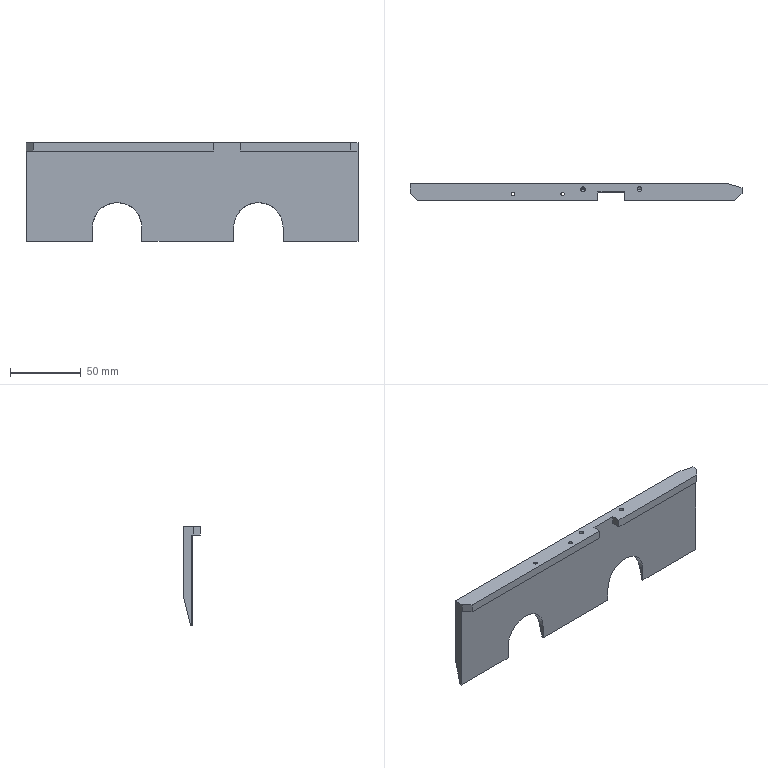Component | SolidWorks | P-SLJ-003-1_P-SLJ-003-001-1 | 1 solid | 38 faces | box 235 x 12 x 70 mm | volume 87007 mm3 | plane 24 | cylinder 10 | cone 4 | commonest cylinder face diameters 3.3 x4 2.5 x4 35 x2 | material A3
build123d program:
from build123d import *

# Parameters (mm, degrees)
EXTRUDE1_DEPTH        = 117.5
EXTRUDE2_REACH        = 247.497
EXTRUDE3_DEPTH        = 138.296
M3_TAPPED_HOLE1_D     = 2.5
M3_TAPPED_HOLE1_DEPTH = 8.5
M3_TAPPED_HOLE1_TIP   = 0.7511
M4_TAPPED_HOLE1_D     = 3.3
M4_TAPPED_HOLE1_DEPTH = 11.5
M4_TAPPED_HOLE1_TIP   = 0.9914
SKETCH9_W             = 19
SKETCH9_H             = 6
EXTRUDE4_DEPTH        = 138.296
CHAMFER1_SIZE         = 5
CHAMFER1_2_SIZE       = 3
CHAMFER1_2_SIZE2      = 10


with BuildPart() as part:
    # Sketch1 → Extrude1 (new, symmetric)
    with BuildSketch(Plane(origin=(0, 0, 0), x_dir=(0, 0, -1), z_dir=(1, 0, 0))):
        Polygon((0, 0), (-6, 0), (-6, 6), (-70, 6), (-70, 12), (0, 12), align=None)
    extrude(amount=EXTRUDE1_DEPTH, both=True)

    # Sketch2 → Extrude2 (cut, up to next)
    with BuildSketch(Plane(origin=(117.5, 0, 0), x_dir=(0, 0, -1), z_dir=(1, 0, 0)), mode=Mode.PRIVATE) as extrude2_sk1:
        Polygon((-70, 7), (-70, 12), (-50, 12), align=None)
    extrude2_tool1 = extrude(extrude2_sk1.sketch, amount=-EXTRUDE2_REACH, mode=Mode.PRIVATE) & part.part
    add(extrude2_tool1.solids().sort_by_distance((117.5, 10.333, 63.333))[0], mode=Mode.SUBTRACT)

    # Sketch3 → Extrude3 (cut, through all)
    with BuildSketch(Plane(origin=(0, 12, 0), x_dir=(1, 0, 0), z_dir=(0, 1, 0))):
        with BuildLine():
            Line((-64.5, -60), (-64.5, -70))
            Line((-64.5, -70), (-29.5, -70))
            Line((-29.5, -70), (-29.5, -60))
            ThreePointArc((-29.5, -60), (-47, -42.5), (-64.5, -60))
        make_face()
        with BuildLine():
            Line((35.5, -60), (35.5, -70))
            Line((35.5, -70), (70.5, -70))
            Line((70.5, -70), (70.5, -60))
            ThreePointArc((70.5, -60), (53, -42.5), (35.5, -60))
        make_face()
    extrude(amount=-EXTRUDE3_DEPTH, mode=Mode.SUBTRACT)

    # M3 Tapped Hole1
    with Locations(Plane(origin=(0, 0, 0), x_dir=(-1, 0, 0), z_dir=(0, 0, -1))):
        with Locations((-44.5, 4.5), (-9.5, 4.5)):
            Hole(M3_TAPPED_HOLE1_D / 2, depth=M3_TAPPED_HOLE1_DEPTH)
            with Locations((0, 0, -(M3_TAPPED_HOLE1_DEPTH + M3_TAPPED_HOLE1_TIP / 2))):  # 118° drill point
                Cone(0, M3_TAPPED_HOLE1_D / 2, M3_TAPPED_HOLE1_TIP, mode=Mode.SUBTRACT)

    # M4 Tapped Hole1
    with Locations(Plane(origin=(0, 0, 0), x_dir=(-1, 0, 0), z_dir=(0, 0, -1))):
        with Locations((5, 8), (45, 8)):
            Hole(M4_TAPPED_HOLE1_D / 2, depth=M4_TAPPED_HOLE1_DEPTH)
            with Locations((0, 0, -(M4_TAPPED_HOLE1_DEPTH + M4_TAPPED_HOLE1_TIP / 2))):  # 118° drill point
                Cone(0, M4_TAPPED_HOLE1_D / 2, M4_TAPPED_HOLE1_TIP, mode=Mode.SUBTRACT)

    # Sketch9 → Extrude4 (cut, through all)
    with BuildSketch(Plane(origin=(0, 0, 0), x_dir=(-1, 0, 0), z_dir=(0, 0, -1))):
        with Locations((25, 3)):
            Rectangle(SKETCH9_W, SKETCH9_H)
    extrude(amount=-EXTRUDE4_DEPTH, mode=Mode.SUBTRACT)

    # Chamfer1
    chamfer1_edges = [part.edges().sort_by_distance(p)[0] for p in [
        (117.5, 0, 3),
        (-117.5, 0, 3),
    ]]
    chamfer(chamfer1_edges, length=CHAMFER1_SIZE)

    # Chamfer1_2
    chamfer1_2_edges = [part.edges().sort_by_distance(p)[0] for p in [
        (-117.5, 12, 25),
    ]]
    chamfer1_2_side = [part.faces().sort_by_distance(p)[0] for p in [
        (-117.5, 8.767, 30.722),
    ]]
    chamfer(chamfer1_2_edges, length=CHAMFER1_2_SIZE, length2=CHAMFER1_2_SIZE2, reference=chamfer1_2_side[0])


solid = part.part

# Placed as in the assembly
solid = solid.moved(Location((-220, -69, 1248.634), (-180, 0, 180)))